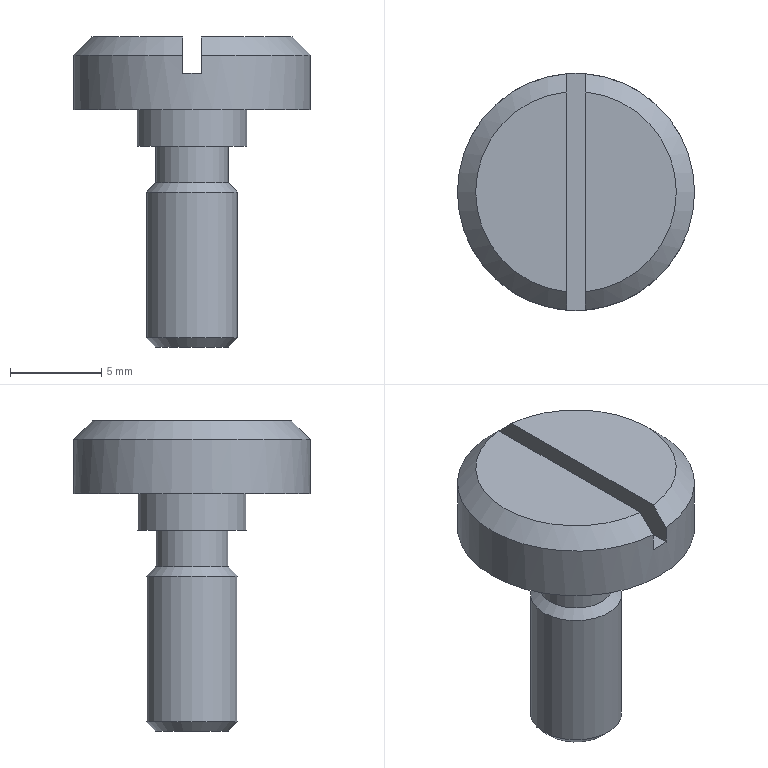Component | NX | SCREW | 1 solid | 16 faces | volume 741 mm3 | plane 8 | cylinder 4 | cone 4 | commonest cylinder face diameters 5 x1 4 x1 6 x1 13 x1